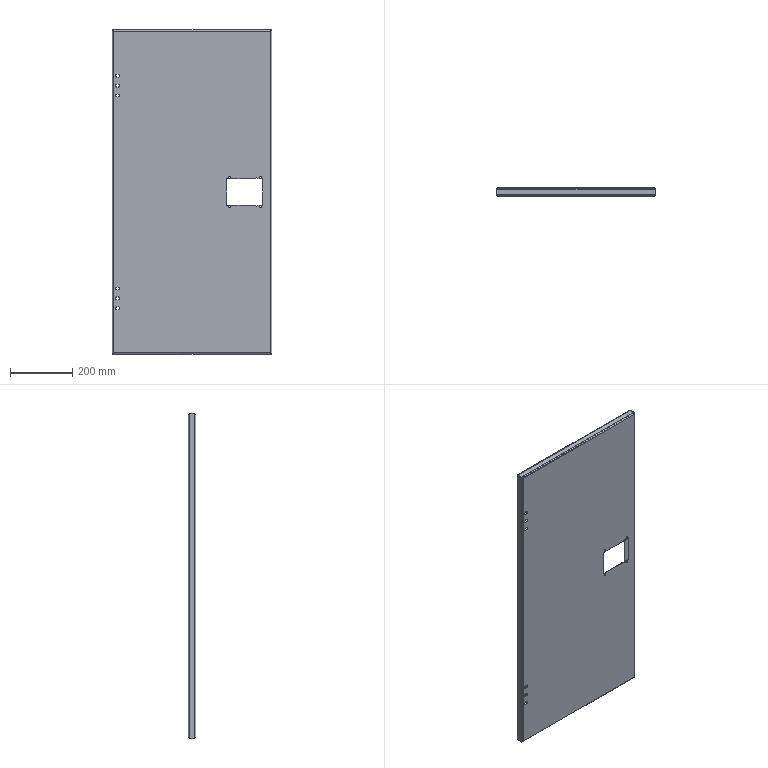Component | SolidWorks | DoorAssembly-1_Door-1 | 1 solid | 136 faces | volume 1315834 mm3 | plane 64 | cylinder 56 | spline 16 | commonest cylinder face diameters 9 x18 7 x10 4 x8 8 x8 10 x8 2 x4 | material Plain Carbon Steel